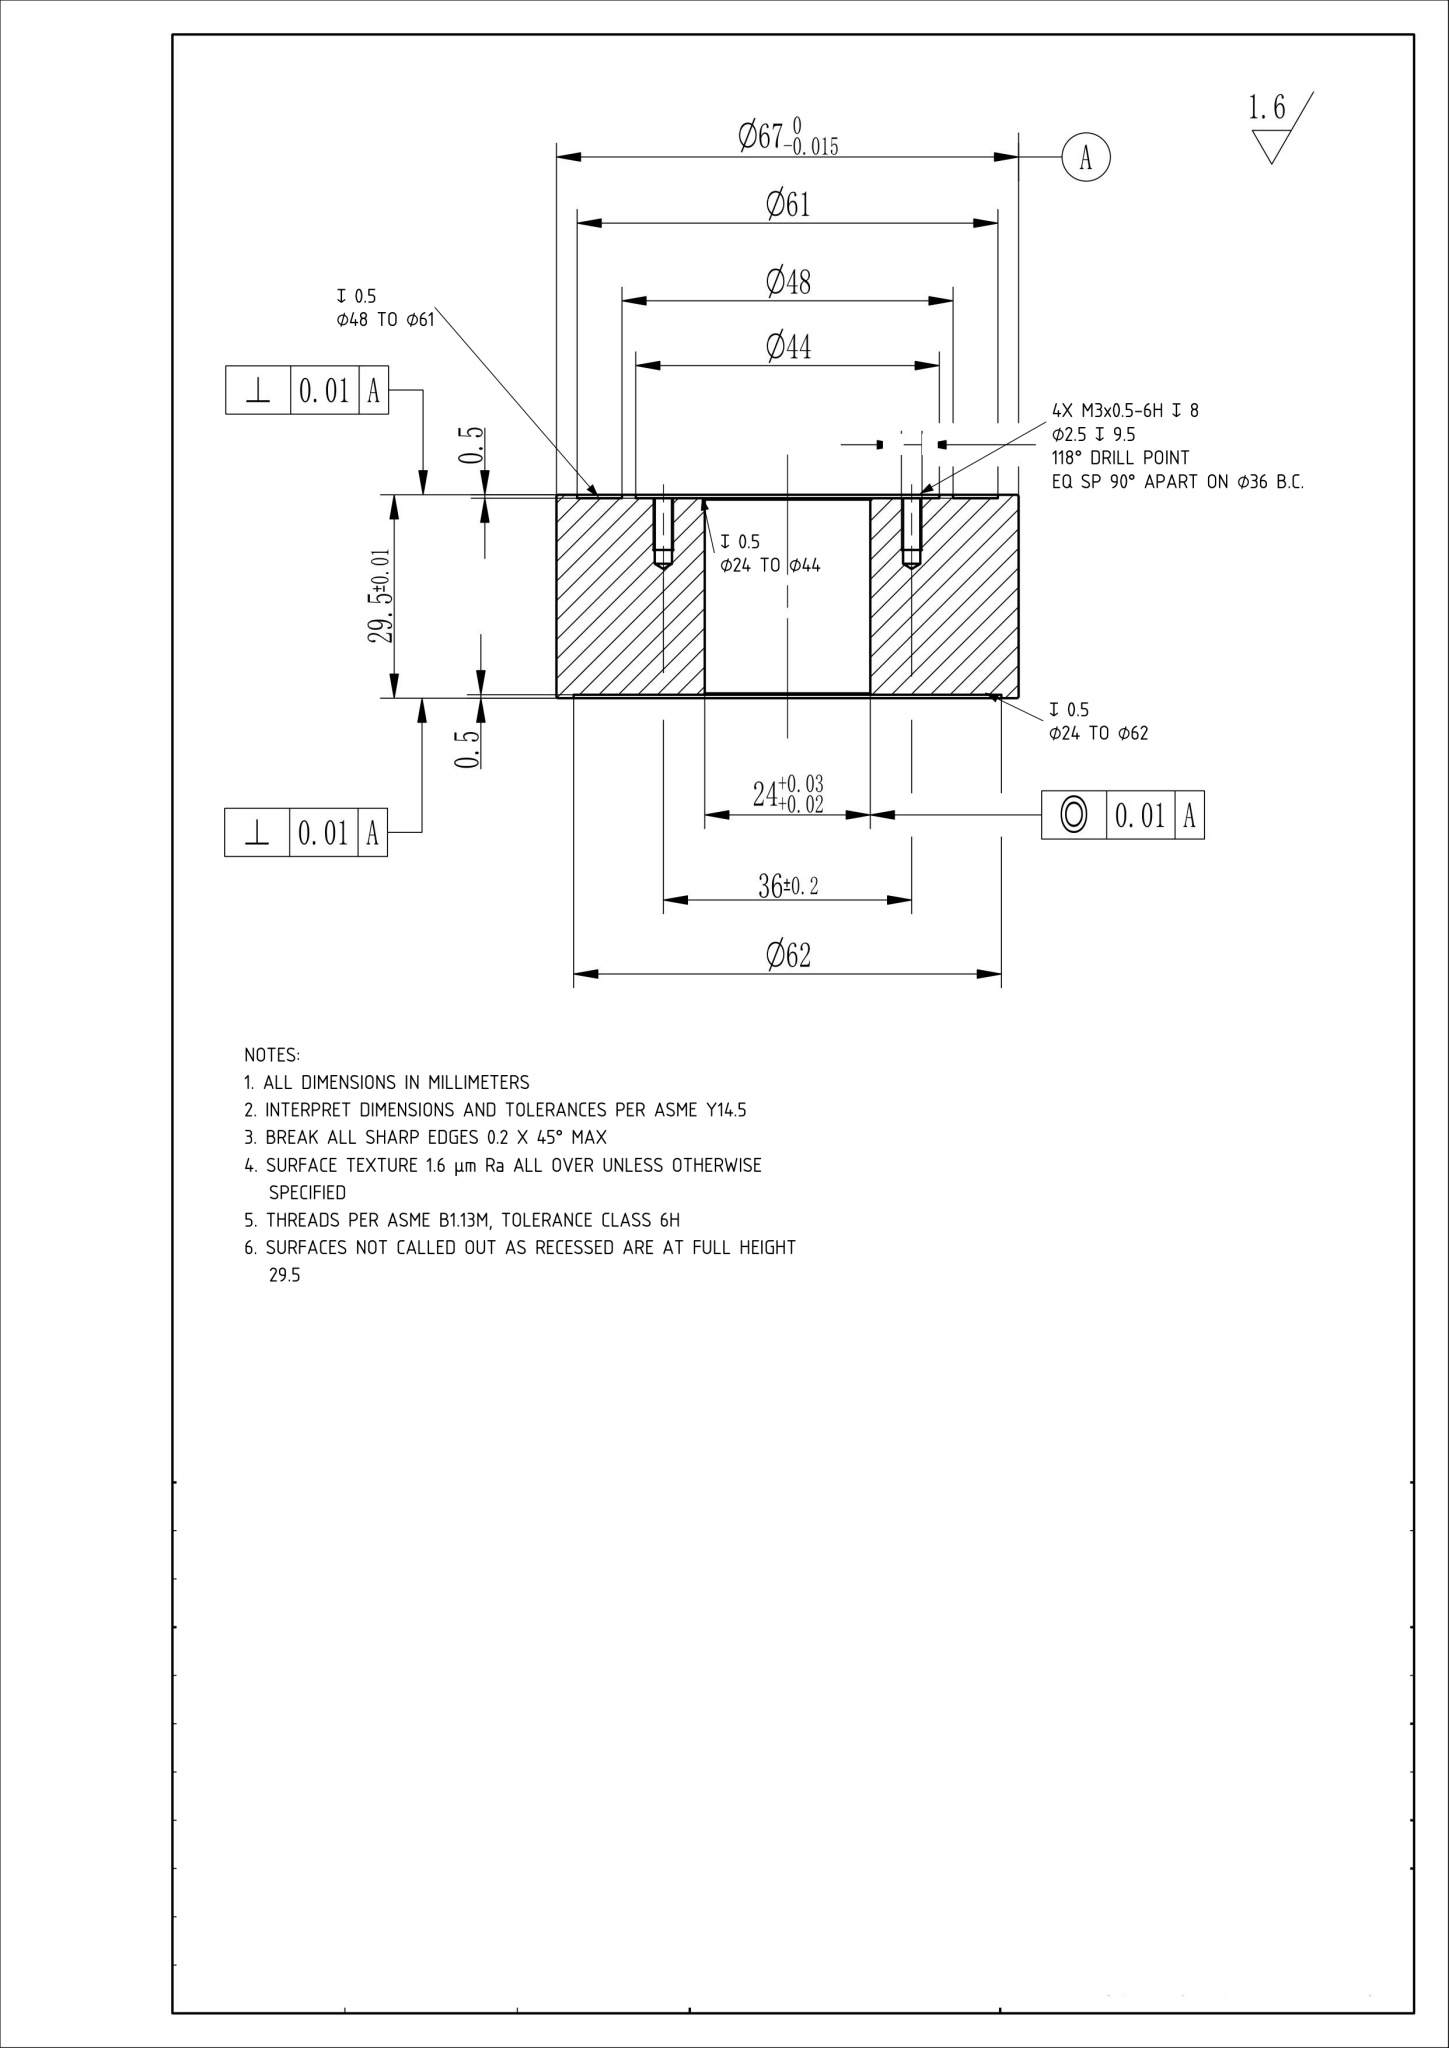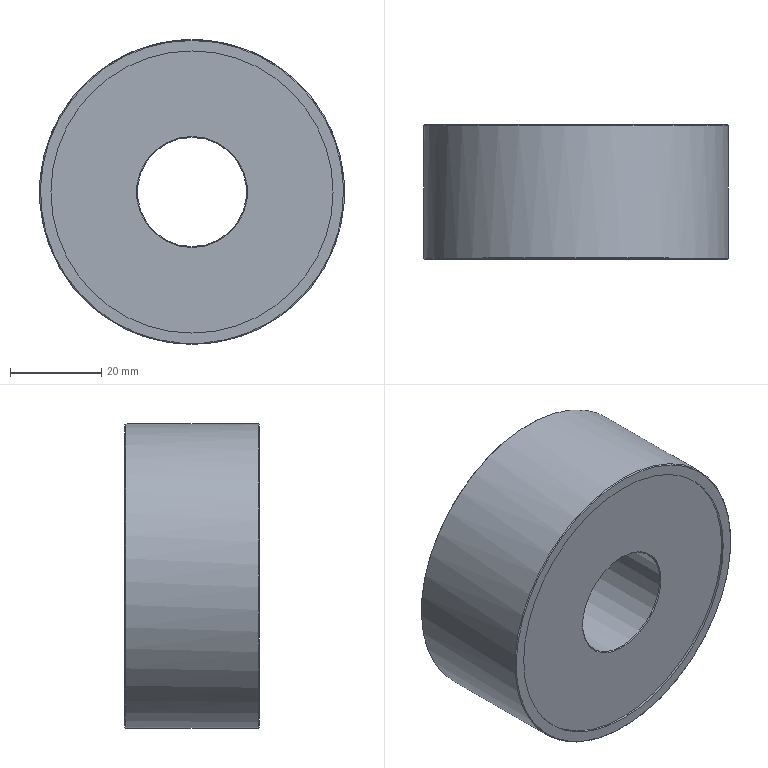Part | NX | mm | 1 solid | 24 faces | box 67 x 29.5 x 67 mm | volume 88085 mm3 | cylinder 10 | cone 8 | plane 6 | commonest cylinder face diameters 2.5 x4 24 x1 67 x1 61 x1 48 x1 44 x1 62 x1
STEP:
#1=CARTESIAN_POINT('',(0.,0.,0.));
#2=DIRECTION('',(0.,0.,1.));
#3=DIRECTION('',(1.,0.,0.));
#4=AXIS2_PLACEMENT_3D('',#1,#2,#3);
#5=(LENGTH_UNIT()NAMED_UNIT(*)SI_UNIT(.MILLI.,.METRE.));
#6=UNCERTAINTY_MEASURE_WITH_UNIT(LENGTH_MEASURE(0.00002),#5,'','');
#7=(NAMED_UNIT(*)PLANE_ANGLE_UNIT()SI_UNIT($,.RADIAN.));
#8=PLANE_ANGLE_MEASURE_WITH_UNIT(PLANE_ANGLE_MEASURE(0.01745),#7);
#9=DIMENSIONAL_EXPONENTS(0.,0.,0.,0.,0.,0.,0.);
#10=(CONVERSION_BASED_UNIT('',#8)NAMED_UNIT(#9)PLANE_ANGLE_UNIT());
#11=(NAMED_UNIT(*)SI_UNIT($,.STERADIAN.)SOLID_ANGLE_UNIT());
#12=(GEOMETRIC_REPRESENTATION_CONTEXT(3)GLOBAL_UNCERTAINTY_ASSIGNED_CONTEXT((#6))GLOBAL_UNIT_ASSIGNED_CONTEXT((#5,#10,#11))REPRESENTATION_CONTEXT('',''));
#13=SHAPE_REPRESENTATION('',(#4),#12);
#14=CARTESIAN_POINT('',(22.,15.25,0.));
#15=VERTEX_POINT('',#14);
#16=CARTESIAN_POINT('',(0.,15.25,0.));
#17=DIRECTION('',(0.,1.,0.));
#18=DIRECTION('',(1.,0.,0.));
#19=AXIS2_PLACEMENT_3D('',#16,#17,#18);
#20=CIRCLE('',#19,22.);
#21=EDGE_CURVE('',#15,#15,#20,.T.);
#22=ORIENTED_EDGE('',*,*,#21,.F.);
#23=EDGE_LOOP('',(#22));
#24=FACE_BOUND('',#23,.T.);
#25=CARTESIAN_POINT('',(24.,15.25,0.));
#26=VERTEX_POINT('',#25);
#27=CARTESIAN_POINT('',(0.,15.25,0.));
#28=DIRECTION('',(0.,1.,0.));
#29=DIRECTION('',(1.,0.,0.));
#30=AXIS2_PLACEMENT_3D('',#27,#28,#29);
#31=CIRCLE('',#30,24.);
#32=EDGE_CURVE('',#26,#26,#31,.T.);
#33=ORIENTED_EDGE('',*,*,#32,.T.);
#34=EDGE_LOOP('',(#33));
#35=FACE_BOUND('',#34,.T.);
#36=CARTESIAN_POINT('',(0.,15.25,12.));
#37=DIRECTION('',(0.,-1.,0.));
#38=DIRECTION('',(0.,0.,-1.));
#39=AXIS2_PLACEMENT_3D('',#36,#37,#38);
#40=PLANE('',#39);
#41=ADVANCED_FACE('',(#24,#35),#40,.F.);
#42=CARTESIAN_POINT('',(31.,-14.25,-0.));
#43=VERTEX_POINT('',#42);
#44=CARTESIAN_POINT('',(0.,-14.25,0.));
#45=DIRECTION('',(0.,-1.,0.));
#46=DIRECTION('',(1.,0.,-0.));
#47=AXIS2_PLACEMENT_3D('',#44,#45,#46);
#48=CIRCLE('',#47,31.);
#49=EDGE_CURVE('',#43,#43,#48,.T.);
#50=ORIENTED_EDGE('',*,*,#49,.F.);
#51=EDGE_LOOP('',(#50));
#52=FACE_BOUND('',#51,.T.);
#53=CARTESIAN_POINT('',(0.,-14.25,33.3));
#54=VERTEX_POINT('',#53);
#55=CARTESIAN_POINT('',(0.,-14.25,0.));
#56=DIRECTION('',(0.,-1.,0.));
#57=DIRECTION('',(0.,0.,1.));
#58=AXIS2_PLACEMENT_3D('',#55,#56,#57);
#59=CIRCLE('',#58,33.3);
#60=EDGE_CURVE('',#54,#54,#59,.T.);
#61=ORIENTED_EDGE('',*,*,#60,.T.);
#62=EDGE_LOOP('',(#61));
#63=FACE_BOUND('',#62,.T.);
#64=CARTESIAN_POINT('',(0.,-14.25,33.5));
#65=DIRECTION('',(0.,1.,0.));
#66=DIRECTION('',(0.,0.,1.));
#67=AXIS2_PLACEMENT_3D('',#64,#65,#66);
#68=PLANE('',#67);
#69=ADVANCED_FACE('',(#52,#63),#68,.F.);
#70=CARTESIAN_POINT('',(0.,-13.55,-12.));
#71=VERTEX_POINT('',#70);
#72=CARTESIAN_POINT('',(0.,-13.55,0.));
#73=DIRECTION('',(0.,-1.,0.));
#74=DIRECTION('',(0.,0.,-1.));
#75=AXIS2_PLACEMENT_3D('',#72,#73,#74);
#76=CIRCLE('',#75,12.);
#77=EDGE_CURVE('',#71,#71,#76,.T.);
#78=ORIENTED_EDGE('',*,*,#77,.T.);
#79=EDGE_LOOP('',(#78));
#80=FACE_BOUND('',#79,.T.);
#81=CARTESIAN_POINT('',(0.,14.55,12.));
#82=VERTEX_POINT('',#81);
#83=CARTESIAN_POINT('',(0.,14.55,0.));
#84=DIRECTION('',(0.,1.,0.));
#85=DIRECTION('',(0.,0.,1.));
#86=AXIS2_PLACEMENT_3D('',#83,#84,#85);
#87=CIRCLE('',#86,12.);
#88=EDGE_CURVE('',#82,#82,#87,.T.);
#89=ORIENTED_EDGE('',*,*,#88,.T.);
#90=EDGE_LOOP('',(#89));
#91=FACE_BOUND('',#90,.T.);
#92=CARTESIAN_POINT('',(0.,0.,0.));
#93=DIRECTION('',(0.,-1.,0.));
#94=DIRECTION('',(0.,0.,-1.));
#95=AXIS2_PLACEMENT_3D('',#92,#93,#94);
#96=CYLINDRICAL_SURFACE('',#95,12.);
#97=ADVANCED_FACE('',(#80,#91),#96,.F.);
#98=CARTESIAN_POINT('',(0.,15.25,-33.3));
#99=VERTEX_POINT('',#98);
#100=CARTESIAN_POINT('',(0.,15.25,0.));
#101=DIRECTION('',(0.,1.,0.));
#102=DIRECTION('',(0.,0.,-1.));
#103=AXIS2_PLACEMENT_3D('',#100,#101,#102);
#104=CIRCLE('',#103,33.3);
#105=EDGE_CURVE('',#99,#99,#104,.T.);
#106=ORIENTED_EDGE('',*,*,#105,.T.);
#107=EDGE_LOOP('',(#106));
#108=FACE_BOUND('',#107,.T.);
#109=CARTESIAN_POINT('',(30.5,15.25,0.));
#110=VERTEX_POINT('',#109);
#111=CARTESIAN_POINT('',(0.,15.25,0.));
#112=DIRECTION('',(0.,1.,0.));
#113=DIRECTION('',(1.,0.,0.));
#114=AXIS2_PLACEMENT_3D('',#111,#112,#113);
#115=CIRCLE('',#114,30.5);
#116=EDGE_CURVE('',#110,#110,#115,.T.);
#117=ORIENTED_EDGE('',*,*,#116,.F.);
#118=EDGE_LOOP('',(#117));
#119=FACE_BOUND('',#118,.T.);
#120=CARTESIAN_POINT('',(0.,15.25,12.));
#121=DIRECTION('',(0.,-1.,0.));
#122=DIRECTION('',(0.,0.,-1.));
#123=AXIS2_PLACEMENT_3D('',#120,#121,#122);
#124=PLANE('',#123);
#125=ADVANCED_FACE('',(#108,#119),#124,.F.);
#126=CARTESIAN_POINT('',(0.,-14.05,33.5));
#127=VERTEX_POINT('',#126);
#128=CARTESIAN_POINT('',(0.,-14.05,0.));
#129=DIRECTION('',(0.,1.,0.));
#130=DIRECTION('',(0.,0.,1.));
#131=AXIS2_PLACEMENT_3D('',#128,#129,#130);
#132=CIRCLE('',#131,33.5);
#133=EDGE_CURVE('',#127,#127,#132,.T.);
#134=ORIENTED_EDGE('',*,*,#133,.T.);
#135=EDGE_LOOP('',(#134));
#136=FACE_BOUND('',#135,.T.);
#137=CARTESIAN_POINT('',(0.,15.05,-33.5));
#138=VERTEX_POINT('',#137);
#139=CARTESIAN_POINT('',(0.,15.05,0.));
#140=DIRECTION('',(0.,-1.,0.));
#141=DIRECTION('',(0.,0.,-1.));
#142=AXIS2_PLACEMENT_3D('',#139,#140,#141);
#143=CIRCLE('',#142,33.5);
#144=EDGE_CURVE('',#138,#138,#143,.T.);
#145=ORIENTED_EDGE('',*,*,#144,.T.);
#146=EDGE_LOOP('',(#145));
#147=FACE_BOUND('',#146,.T.);
#148=CARTESIAN_POINT('',(0.,0.,0.));
#149=DIRECTION('',(0.,-1.,0.));
#150=DIRECTION('',(0.,0.,-1.));
#151=AXIS2_PLACEMENT_3D('',#148,#149,#150);
#152=CYLINDRICAL_SURFACE('',#151,33.5);
#153=ADVANCED_FACE('',(#136,#147),#152,.T.);
#154=CARTESIAN_POINT('',(30.5,14.75,0.));
#155=VERTEX_POINT('',#154);
#156=CARTESIAN_POINT('',(0.,14.75,0.));
#157=DIRECTION('',(0.,-1.,0.));
#158=DIRECTION('',(1.,0.,0.));
#159=AXIS2_PLACEMENT_3D('',#156,#157,#158);
#160=CIRCLE('',#159,30.5);
#161=EDGE_CURVE('',#155,#155,#160,.T.);
#162=ORIENTED_EDGE('',*,*,#161,.T.);
#163=EDGE_LOOP('',(#162));
#164=FACE_BOUND('',#163,.T.);
#165=ORIENTED_EDGE('',*,*,#116,.T.);
#166=EDGE_LOOP('',(#165));
#167=FACE_BOUND('',#166,.T.);
#168=CARTESIAN_POINT('',(0.,14.75,0.));
#169=DIRECTION('',(0.,1.,0.));
#170=DIRECTION('',(0.,0.,1.));
#171=AXIS2_PLACEMENT_3D('',#168,#169,#170);
#172=CYLINDRICAL_SURFACE('',#171,30.5);
#173=ADVANCED_FACE('',(#164,#167),#172,.F.);
#174=CARTESIAN_POINT('',(24.,14.75,0.));
#175=VERTEX_POINT('',#174);
#176=CARTESIAN_POINT('',(0.,14.75,0.));
#177=DIRECTION('',(0.,-1.,0.));
#178=DIRECTION('',(1.,0.,0.));
#179=AXIS2_PLACEMENT_3D('',#176,#177,#178);
#180=CIRCLE('',#179,24.);
#181=EDGE_CURVE('',#175,#175,#180,.T.);
#182=ORIENTED_EDGE('',*,*,#181,.F.);
#183=EDGE_LOOP('',(#182));
#184=FACE_BOUND('',#183,.T.);
#185=ORIENTED_EDGE('',*,*,#32,.F.);
#186=EDGE_LOOP('',(#185));
#187=FACE_BOUND('',#186,.T.);
#188=CARTESIAN_POINT('',(0.,14.75,0.));
#189=DIRECTION('',(0.,1.,0.));
#190=DIRECTION('',(0.,0.,1.));
#191=AXIS2_PLACEMENT_3D('',#188,#189,#190);
#192=CYLINDRICAL_SURFACE('',#191,24.);
#193=ADVANCED_FACE('',(#184,#187),#192,.T.);
#194=ORIENTED_EDGE('',*,*,#161,.F.);
#195=EDGE_LOOP('',(#194));
#196=FACE_BOUND('',#195,.T.);
#197=ORIENTED_EDGE('',*,*,#181,.T.);
#198=EDGE_LOOP('',(#197));
#199=FACE_BOUND('',#198,.T.);
#200=CARTESIAN_POINT('',(0.,14.75,0.));
#201=DIRECTION('',(0.,1.,0.));
#202=DIRECTION('',(0.,0.,1.));
#203=AXIS2_PLACEMENT_3D('',#200,#201,#202);
#204=PLANE('',#203);
#205=ADVANCED_FACE('',(#196,#199),#204,.T.);
#206=CARTESIAN_POINT('',(0.,14.75,12.2));
#207=VERTEX_POINT('',#206);
#208=CARTESIAN_POINT('',(0.,14.75,0.));
#209=DIRECTION('',(0.,-1.,0.));
#210=DIRECTION('',(0.,0.,1.));
#211=AXIS2_PLACEMENT_3D('',#208,#209,#210);
#212=CIRCLE('',#211,12.2);
#213=EDGE_CURVE('',#207,#207,#212,.T.);
#214=ORIENTED_EDGE('',*,*,#213,.T.);
#215=EDGE_LOOP('',(#214));
#216=FACE_BOUND('',#215,.T.);
#217=CARTESIAN_POINT('',(22.,14.75,0.));
#218=VERTEX_POINT('',#217);
#219=CARTESIAN_POINT('',(0.,14.75,0.));
#220=DIRECTION('',(0.,-1.,0.));
#221=DIRECTION('',(1.,0.,0.));
#222=AXIS2_PLACEMENT_3D('',#219,#220,#221);
#223=CIRCLE('',#222,22.);
#224=EDGE_CURVE('',#218,#218,#223,.T.);
#225=ORIENTED_EDGE('',*,*,#224,.F.);
#226=EDGE_LOOP('',(#225));
#227=FACE_BOUND('',#226,.T.);
#228=CARTESIAN_POINT('',(-0.,14.75,19.25));
#229=VERTEX_POINT('',#228);
#230=CARTESIAN_POINT('',(-0.,14.75,18.));
#231=DIRECTION('',(0.,-1.,0.));
#232=DIRECTION('',(0.,0.,1.));
#233=AXIS2_PLACEMENT_3D('',#230,#231,#232);
#234=CIRCLE('',#233,1.25);
#235=EDGE_CURVE('',#229,#229,#234,.T.);
#236=ORIENTED_EDGE('',*,*,#235,.T.);
#237=EDGE_LOOP('',(#236));
#238=FACE_BOUND('',#237,.T.);
#239=CARTESIAN_POINT('',(-18.,14.75,1.25));
#240=VERTEX_POINT('',#239);
#241=CARTESIAN_POINT('',(-18.,14.75,0.));
#242=DIRECTION('',(0.,-1.,0.));
#243=DIRECTION('',(0.,0.,1.));
#244=AXIS2_PLACEMENT_3D('',#241,#242,#243);
#245=CIRCLE('',#244,1.25);
#246=EDGE_CURVE('',#240,#240,#245,.T.);
#247=ORIENTED_EDGE('',*,*,#246,.T.);
#248=EDGE_LOOP('',(#247));
#249=FACE_BOUND('',#248,.T.);
#250=CARTESIAN_POINT('',(0.,14.75,-16.75));
#251=VERTEX_POINT('',#250);
#252=CARTESIAN_POINT('',(0.,14.75,-18.));
#253=DIRECTION('',(0.,-1.,0.));
#254=DIRECTION('',(0.,0.,1.));
#255=AXIS2_PLACEMENT_3D('',#252,#253,#254);
#256=CIRCLE('',#255,1.25);
#257=EDGE_CURVE('',#251,#251,#256,.T.);
#258=ORIENTED_EDGE('',*,*,#257,.T.);
#259=EDGE_LOOP('',(#258));
#260=FACE_BOUND('',#259,.T.);
#261=CARTESIAN_POINT('',(18.,14.75,1.25));
#262=VERTEX_POINT('',#261);
#263=CARTESIAN_POINT('',(18.,14.75,0.));
#264=DIRECTION('',(0.,-1.,0.));
#265=DIRECTION('',(0.,0.,1.));
#266=AXIS2_PLACEMENT_3D('',#263,#264,#265);
#267=CIRCLE('',#266,1.25);
#268=EDGE_CURVE('',#262,#262,#267,.T.);
#269=ORIENTED_EDGE('',*,*,#268,.T.);
#270=EDGE_LOOP('',(#269));
#271=FACE_BOUND('',#270,.T.);
#272=CARTESIAN_POINT('',(0.,14.75,0.));
#273=DIRECTION('',(0.,1.,0.));
#274=DIRECTION('',(0.,0.,1.));
#275=AXIS2_PLACEMENT_3D('',#272,#273,#274);
#276=PLANE('',#275);
#277=ADVANCED_FACE('',(#216,#227,#238,#249,#260,#271),#276,.T.);
#278=ORIENTED_EDGE('',*,*,#224,.T.);
#279=EDGE_LOOP('',(#278));
#280=FACE_BOUND('',#279,.T.);
#281=ORIENTED_EDGE('',*,*,#21,.T.);
#282=EDGE_LOOP('',(#281));
#283=FACE_BOUND('',#282,.T.);
#284=CARTESIAN_POINT('',(0.,14.75,0.));
#285=DIRECTION('',(0.,1.,0.));
#286=DIRECTION('',(0.,0.,1.));
#287=AXIS2_PLACEMENT_3D('',#284,#285,#286);
#288=CYLINDRICAL_SURFACE('',#287,22.);
#289=ADVANCED_FACE('',(#280,#283),#288,.F.);
#290=CARTESIAN_POINT('',(-18.,5.25,-1.25));
#291=VERTEX_POINT('',#290);
#292=CARTESIAN_POINT('',(-18.,5.25,0.));
#293=DIRECTION('',(0.,1.,0.));
#294=DIRECTION('',(0.,0.,-1.));
#295=AXIS2_PLACEMENT_3D('',#292,#293,#294);
#296=CIRCLE('',#295,1.25);
#297=EDGE_CURVE('',#291,#291,#296,.T.);
#298=ORIENTED_EDGE('',*,*,#297,.T.);
#299=EDGE_LOOP('',(#298));
#300=FACE_BOUND('',#299,.T.);
#301=CARTESIAN_POINT('',(-18.,4.499,0.));
#302=VERTEX_POINT('',#301);
#303=VERTEX_LOOP('',#302);
#304=FACE_BOUND('',#303,.T.);
#305=CARTESIAN_POINT('',(-18.,5.25,0.));
#306=DIRECTION('',(0.,1.,0.));
#307=DIRECTION('',(0.,-0.,1.));
#308=AXIS2_PLACEMENT_3D('',#305,#306,#307);
#309=CONICAL_SURFACE('',#308,1.25,59.);
#310=ADVANCED_FACE('',(#300,#304),#309,.F.);
#311=ORIENTED_EDGE('',*,*,#297,.F.);
#312=EDGE_LOOP('',(#311));
#313=FACE_BOUND('',#312,.T.);
#314=ORIENTED_EDGE('',*,*,#246,.F.);
#315=EDGE_LOOP('',(#314));
#316=FACE_BOUND('',#315,.T.);
#317=CARTESIAN_POINT('',(-18.,15.25,0.));
#318=DIRECTION('',(0.,-1.,0.));
#319=DIRECTION('',(0.,0.,-1.));
#320=AXIS2_PLACEMENT_3D('',#317,#318,#319);
#321=CYLINDRICAL_SURFACE('',#320,1.25);
#322=ADVANCED_FACE('',(#313,#316),#321,.F.);
#323=CARTESIAN_POINT('',(0.,5.25,-19.25));
#324=VERTEX_POINT('',#323);
#325=CARTESIAN_POINT('',(0.,5.25,-18.));
#326=DIRECTION('',(0.,1.,0.));
#327=DIRECTION('',(0.,0.,-1.));
#328=AXIS2_PLACEMENT_3D('',#325,#326,#327);
#329=CIRCLE('',#328,1.25);
#330=EDGE_CURVE('',#324,#324,#329,.T.);
#331=ORIENTED_EDGE('',*,*,#330,.T.);
#332=EDGE_LOOP('',(#331));
#333=FACE_BOUND('',#332,.T.);
#334=CARTESIAN_POINT('',(0.,4.499,-18.));
#335=VERTEX_POINT('',#334);
#336=VERTEX_LOOP('',#335);
#337=FACE_BOUND('',#336,.T.);
#338=CARTESIAN_POINT('',(0.,5.25,-18.));
#339=DIRECTION('',(0.,1.,0.));
#340=DIRECTION('',(0.,-0.,1.));
#341=AXIS2_PLACEMENT_3D('',#338,#339,#340);
#342=CONICAL_SURFACE('',#341,1.25,59.);
#343=ADVANCED_FACE('',(#333,#337),#342,.F.);
#344=ORIENTED_EDGE('',*,*,#330,.F.);
#345=EDGE_LOOP('',(#344));
#346=FACE_BOUND('',#345,.T.);
#347=ORIENTED_EDGE('',*,*,#257,.F.);
#348=EDGE_LOOP('',(#347));
#349=FACE_BOUND('',#348,.T.);
#350=CARTESIAN_POINT('',(0.,15.25,-18.));
#351=DIRECTION('',(0.,-1.,0.));
#352=DIRECTION('',(0.,0.,-1.));
#353=AXIS2_PLACEMENT_3D('',#350,#351,#352);
#354=CYLINDRICAL_SURFACE('',#353,1.25);
#355=ADVANCED_FACE('',(#346,#349),#354,.F.);
#356=CARTESIAN_POINT('',(18.,5.25,-1.25));
#357=VERTEX_POINT('',#356);
#358=CARTESIAN_POINT('',(18.,5.25,0.));
#359=DIRECTION('',(0.,1.,0.));
#360=DIRECTION('',(0.,0.,-1.));
#361=AXIS2_PLACEMENT_3D('',#358,#359,#360);
#362=CIRCLE('',#361,1.25);
#363=EDGE_CURVE('',#357,#357,#362,.T.);
#364=ORIENTED_EDGE('',*,*,#363,.T.);
#365=EDGE_LOOP('',(#364));
#366=FACE_BOUND('',#365,.T.);
#367=CARTESIAN_POINT('',(18.,4.499,0.));
#368=VERTEX_POINT('',#367);
#369=VERTEX_LOOP('',#368);
#370=FACE_BOUND('',#369,.T.);
#371=CARTESIAN_POINT('',(18.,5.25,0.));
#372=DIRECTION('',(0.,1.,0.));
#373=DIRECTION('',(0.,-0.,1.));
#374=AXIS2_PLACEMENT_3D('',#371,#372,#373);
#375=CONICAL_SURFACE('',#374,1.25,59.);
#376=ADVANCED_FACE('',(#366,#370),#375,.F.);
#377=ORIENTED_EDGE('',*,*,#363,.F.);
#378=EDGE_LOOP('',(#377));
#379=FACE_BOUND('',#378,.T.);
#380=ORIENTED_EDGE('',*,*,#268,.F.);
#381=EDGE_LOOP('',(#380));
#382=FACE_BOUND('',#381,.T.);
#383=CARTESIAN_POINT('',(18.,15.25,0.));
#384=DIRECTION('',(0.,-1.,0.));
#385=DIRECTION('',(0.,0.,-1.));
#386=AXIS2_PLACEMENT_3D('',#383,#384,#385);
#387=CYLINDRICAL_SURFACE('',#386,1.25);
#388=ADVANCED_FACE('',(#379,#382),#387,.F.);
#389=CARTESIAN_POINT('',(-0.,5.25,16.75));
#390=VERTEX_POINT('',#389);
#391=CARTESIAN_POINT('',(-0.,5.25,18.));
#392=DIRECTION('',(0.,1.,0.));
#393=DIRECTION('',(0.,0.,-1.));
#394=AXIS2_PLACEMENT_3D('',#391,#392,#393);
#395=CIRCLE('',#394,1.25);
#396=EDGE_CURVE('',#390,#390,#395,.T.);
#397=ORIENTED_EDGE('',*,*,#396,.T.);
#398=EDGE_LOOP('',(#397));
#399=FACE_BOUND('',#398,.T.);
#400=CARTESIAN_POINT('',(-0.,4.499,18.));
#401=VERTEX_POINT('',#400);
#402=VERTEX_LOOP('',#401);
#403=FACE_BOUND('',#402,.T.);
#404=CARTESIAN_POINT('',(-0.,5.25,18.));
#405=DIRECTION('',(0.,1.,0.));
#406=DIRECTION('',(0.,-0.,1.));
#407=AXIS2_PLACEMENT_3D('',#404,#405,#406);
#408=CONICAL_SURFACE('',#407,1.25,59.);
#409=ADVANCED_FACE('',(#399,#403),#408,.F.);
#410=ORIENTED_EDGE('',*,*,#396,.F.);
#411=EDGE_LOOP('',(#410));
#412=FACE_BOUND('',#411,.T.);
#413=ORIENTED_EDGE('',*,*,#235,.F.);
#414=EDGE_LOOP('',(#413));
#415=FACE_BOUND('',#414,.T.);
#416=CARTESIAN_POINT('',(-0.,15.25,18.));
#417=DIRECTION('',(0.,-1.,0.));
#418=DIRECTION('',(0.,0.,-1.));
#419=AXIS2_PLACEMENT_3D('',#416,#417,#418);
#420=CYLINDRICAL_SURFACE('',#419,1.25);
#421=ADVANCED_FACE('',(#412,#415),#420,.F.);
#422=ORIENTED_EDGE('',*,*,#213,.F.);
#423=EDGE_LOOP('',(#422));
#424=FACE_BOUND('',#423,.T.);
#425=ORIENTED_EDGE('',*,*,#88,.F.);
#426=EDGE_LOOP('',(#425));
#427=FACE_BOUND('',#426,.T.);
#428=CARTESIAN_POINT('',(0.,14.55,0.));
#429=DIRECTION('',(0.,1.,0.));
#430=DIRECTION('',(0.,0.,1.));
#431=AXIS2_PLACEMENT_3D('',#428,#429,#430);
#432=CONICAL_SURFACE('',#431,12.,45.);
#433=ADVANCED_FACE('',(#424,#427),#432,.F.);
#434=ORIENTED_EDGE('',*,*,#133,.F.);
#435=EDGE_LOOP('',(#434));
#436=FACE_BOUND('',#435,.T.);
#437=ORIENTED_EDGE('',*,*,#60,.F.);
#438=EDGE_LOOP('',(#437));
#439=FACE_BOUND('',#438,.T.);
#440=CARTESIAN_POINT('',(0.,-14.25,0.));
#441=DIRECTION('',(0.,1.,0.));
#442=DIRECTION('',(0.,0.,1.));
#443=AXIS2_PLACEMENT_3D('',#440,#441,#442);
#444=CONICAL_SURFACE('',#443,33.3,45.);
#445=ADVANCED_FACE('',(#436,#439),#444,.T.);
#446=ORIENTED_EDGE('',*,*,#105,.F.);
#447=EDGE_LOOP('',(#446));
#448=FACE_BOUND('',#447,.T.);
#449=ORIENTED_EDGE('',*,*,#144,.F.);
#450=EDGE_LOOP('',(#449));
#451=FACE_BOUND('',#450,.T.);
#452=CARTESIAN_POINT('',(0.,15.05,0.));
#453=DIRECTION('',(0.,-1.,0.));
#454=DIRECTION('',(0.,0.,-1.));
#455=AXIS2_PLACEMENT_3D('',#452,#453,#454);
#456=CONICAL_SURFACE('',#455,33.5,45.);
#457=ADVANCED_FACE('',(#448,#451),#456,.T.);
#458=CARTESIAN_POINT('',(31.,-13.75,-0.));
#459=VERTEX_POINT('',#458);
#460=CARTESIAN_POINT('',(0.,-13.75,0.));
#461=DIRECTION('',(0.,1.,0.));
#462=DIRECTION('',(1.,0.,-0.));
#463=AXIS2_PLACEMENT_3D('',#460,#461,#462);
#464=CIRCLE('',#463,31.);
#465=EDGE_CURVE('',#459,#459,#464,.T.);
#466=ORIENTED_EDGE('',*,*,#465,.T.);
#467=EDGE_LOOP('',(#466));
#468=FACE_BOUND('',#467,.T.);
#469=ORIENTED_EDGE('',*,*,#49,.T.);
#470=EDGE_LOOP('',(#469));
#471=FACE_BOUND('',#470,.T.);
#472=CARTESIAN_POINT('',(0.,-13.75,0.));
#473=DIRECTION('',(0.,-1.,0.));
#474=DIRECTION('',(0.,0.,-1.));
#475=AXIS2_PLACEMENT_3D('',#472,#473,#474);
#476=CYLINDRICAL_SURFACE('',#475,31.);
#477=ADVANCED_FACE('',(#468,#471),#476,.F.);
#478=CARTESIAN_POINT('',(0.,-13.75,-12.2));
#479=VERTEX_POINT('',#478);
#480=CARTESIAN_POINT('',(0.,-13.75,0.));
#481=DIRECTION('',(0.,1.,0.));
#482=DIRECTION('',(0.,0.,-1.));
#483=AXIS2_PLACEMENT_3D('',#480,#481,#482);
#484=CIRCLE('',#483,12.2);
#485=EDGE_CURVE('',#479,#479,#484,.T.);
#486=ORIENTED_EDGE('',*,*,#485,.T.);
#487=EDGE_LOOP('',(#486));
#488=FACE_BOUND('',#487,.T.);
#489=ORIENTED_EDGE('',*,*,#465,.F.);
#490=EDGE_LOOP('',(#489));
#491=FACE_BOUND('',#490,.T.);
#492=CARTESIAN_POINT('',(0.,-13.75,0.));
#493=DIRECTION('',(0.,-1.,0.));
#494=DIRECTION('',(0.,0.,-1.));
#495=AXIS2_PLACEMENT_3D('',#492,#493,#494);
#496=PLANE('',#495);
#497=ADVANCED_FACE('',(#488,#491),#496,.T.);
#498=ORIENTED_EDGE('',*,*,#485,.F.);
#499=EDGE_LOOP('',(#498));
#500=FACE_BOUND('',#499,.T.);
#501=ORIENTED_EDGE('',*,*,#77,.F.);
#502=EDGE_LOOP('',(#501));
#503=FACE_BOUND('',#502,.T.);
#504=CARTESIAN_POINT('',(0.,-13.55,0.));
#505=DIRECTION('',(0.,-1.,0.));
#506=DIRECTION('',(0.,0.,-1.));
#507=AXIS2_PLACEMENT_3D('',#504,#505,#506);
#508=CONICAL_SURFACE('',#507,12.,45.);
#509=ADVANCED_FACE('',(#500,#503),#508,.F.);
#510=CLOSED_SHELL('',(#41,#69,#97,#125,#153,#173,#193,#205,#277,#289,#310,#322,#343,#355,#376,#388,#409,#421,#433,#445,#457,#477,#497,#509));
#511=MANIFOLD_SOLID_BREP('',#510);
#512=ADVANCED_BREP_SHAPE_REPRESENTATION('',(#511),#12);
#513=SHAPE_REPRESENTATION_RELATIONSHIP('','',#13,#512);
#514=PRESENTATION_LAYER_ASSIGNMENT('','',(#511));
#515=COLOUR_RGB('',1.,0.6,0.);
#516=FILL_AREA_STYLE_COLOUR('',#515);
#517=FILL_AREA_STYLE('',(#516));
#518=SURFACE_STYLE_FILL_AREA(#517);
#519=SURFACE_SIDE_STYLE('',(#518));
#520=SURFACE_STYLE_USAGE(.BOTH.,#519);
#521=PRESENTATION_STYLE_ASSIGNMENT((#520));
#522=STYLED_ITEM('',(#521),#511);
#523=MECHANICAL_DESIGN_GEOMETRIC_PRESENTATION_REPRESENTATION('',(#522),#12);